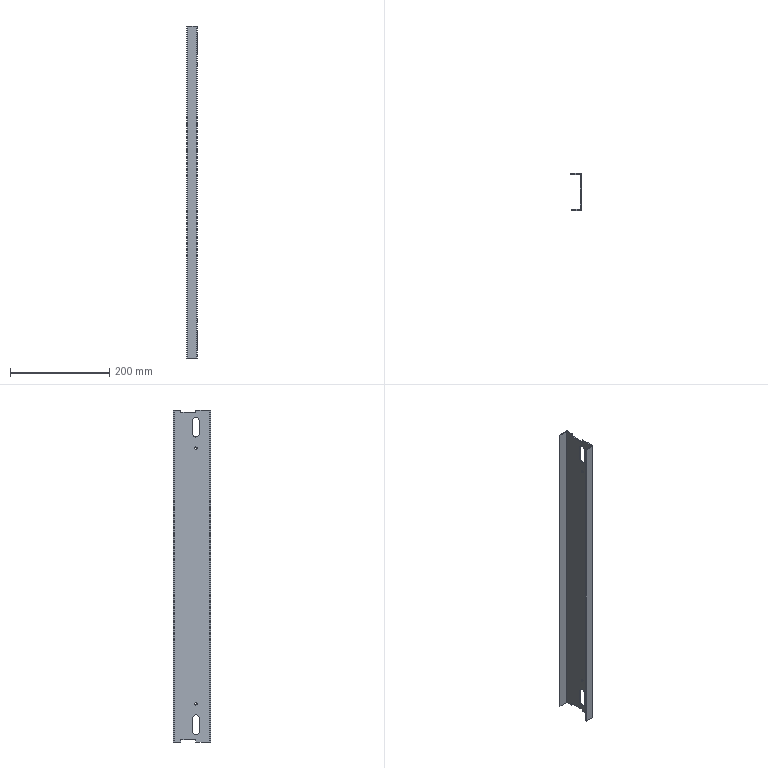Component | SolidWorks | CabinetFrameWeldmentDrawingPG50-01-00-1_BaseWeldingDrawingPG50-05-1_BaseWeldment2(PG50-05-102-1 | 1 solid | 44 faces | volume 147338 mm3 | plane 30 | cylinder 14 | commonest cylinder face diameters 5 x4 13.004 x3 12.7 x3 4.2 x2 0.2 x2 | material AISI 1045 Steel, cold drawn